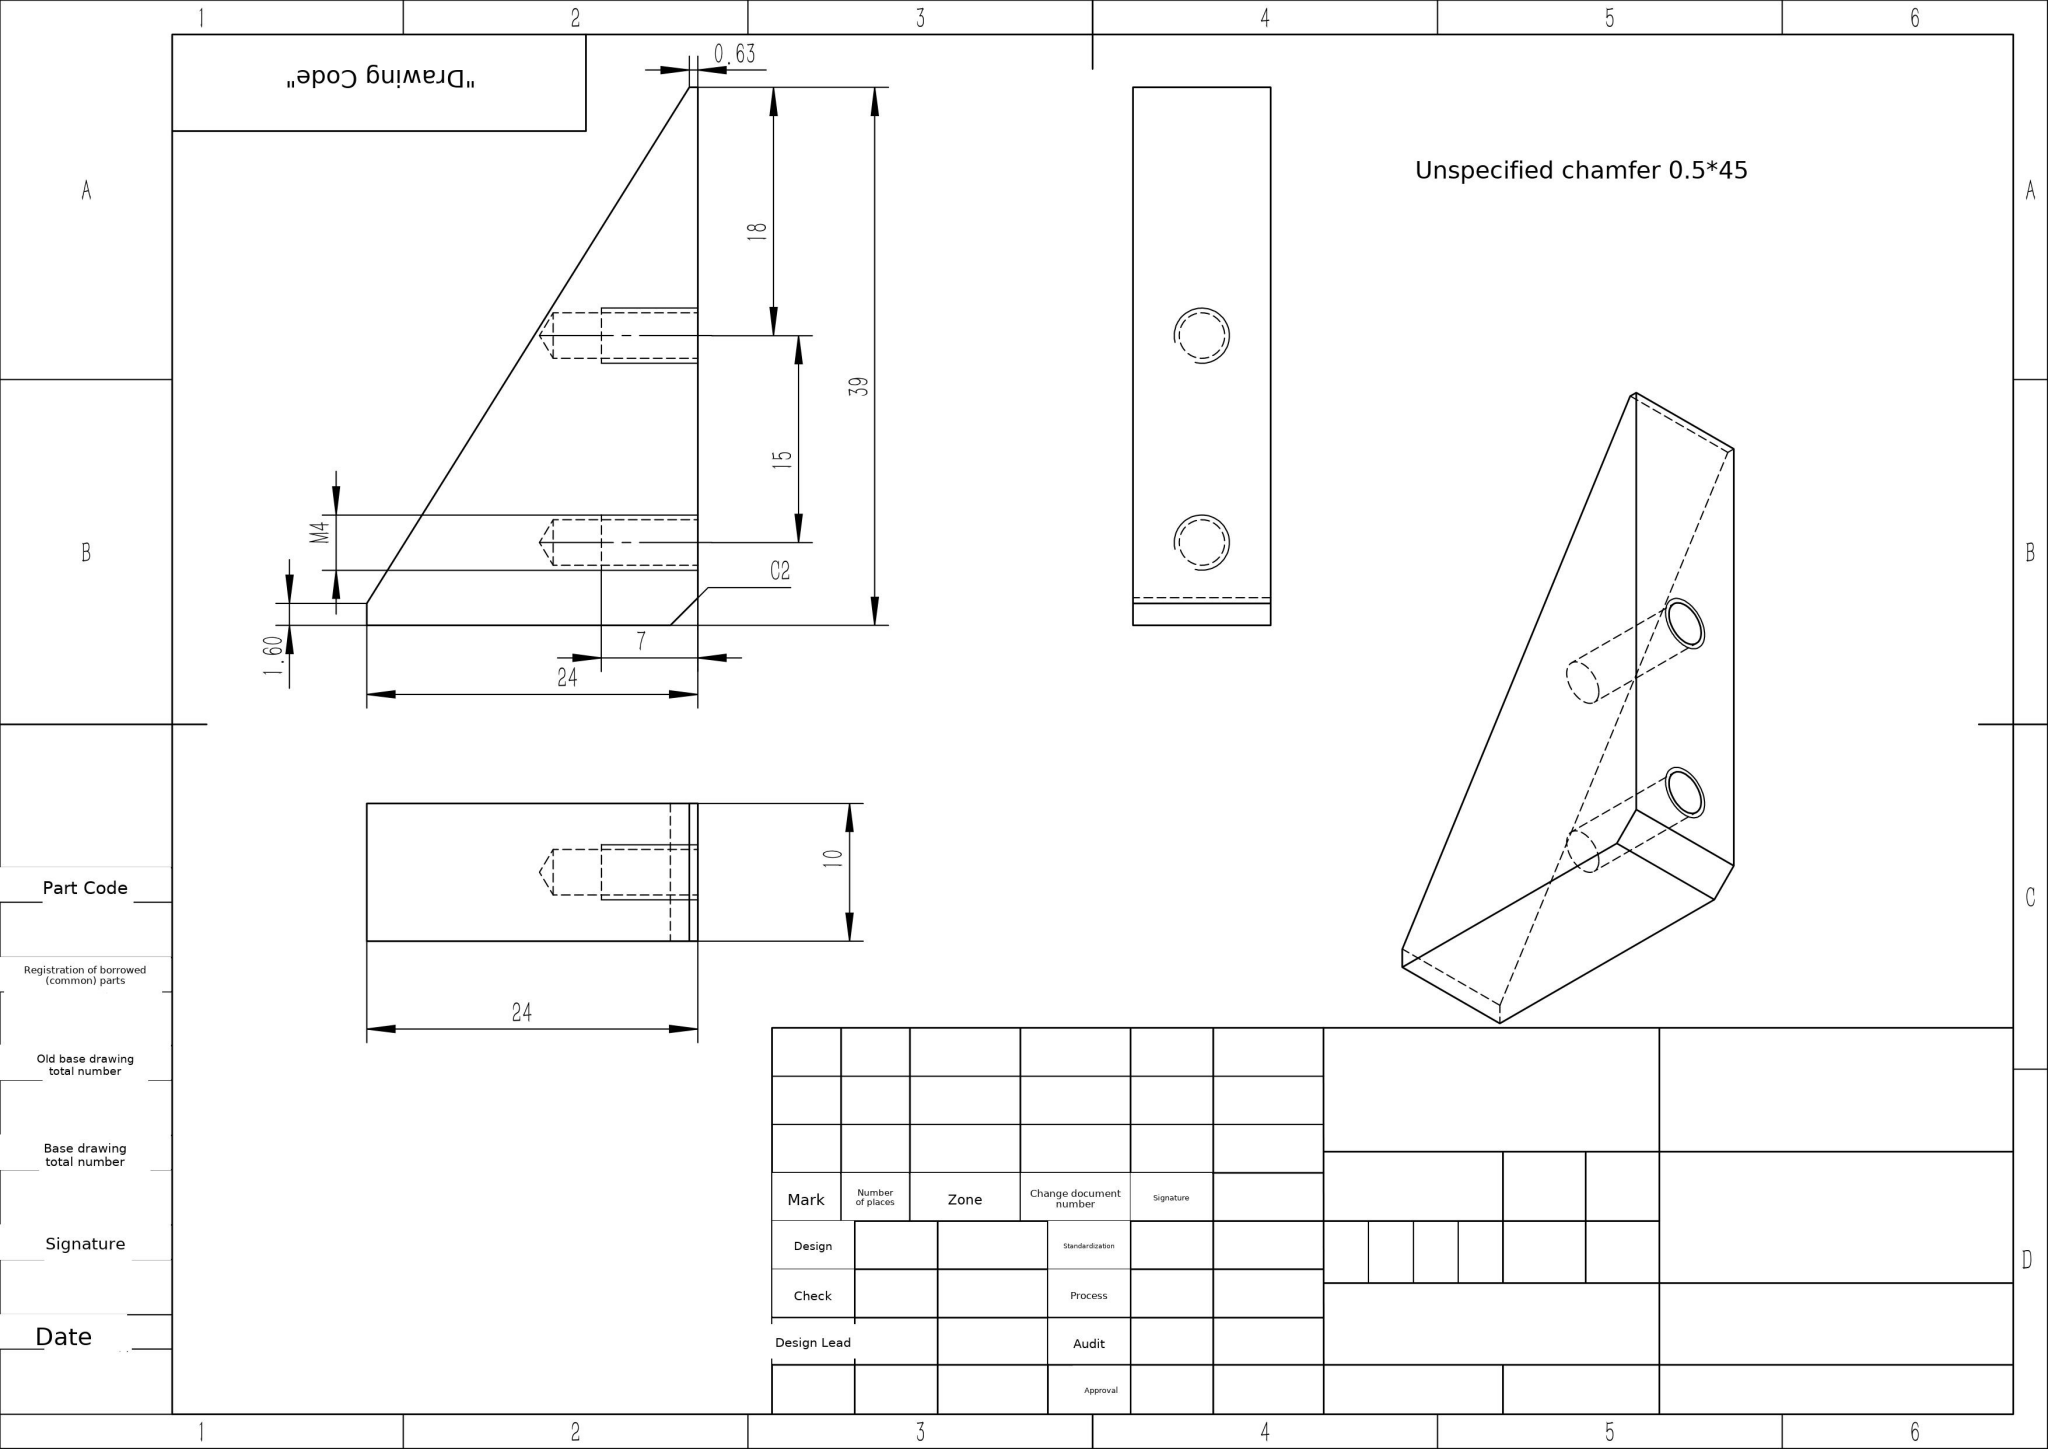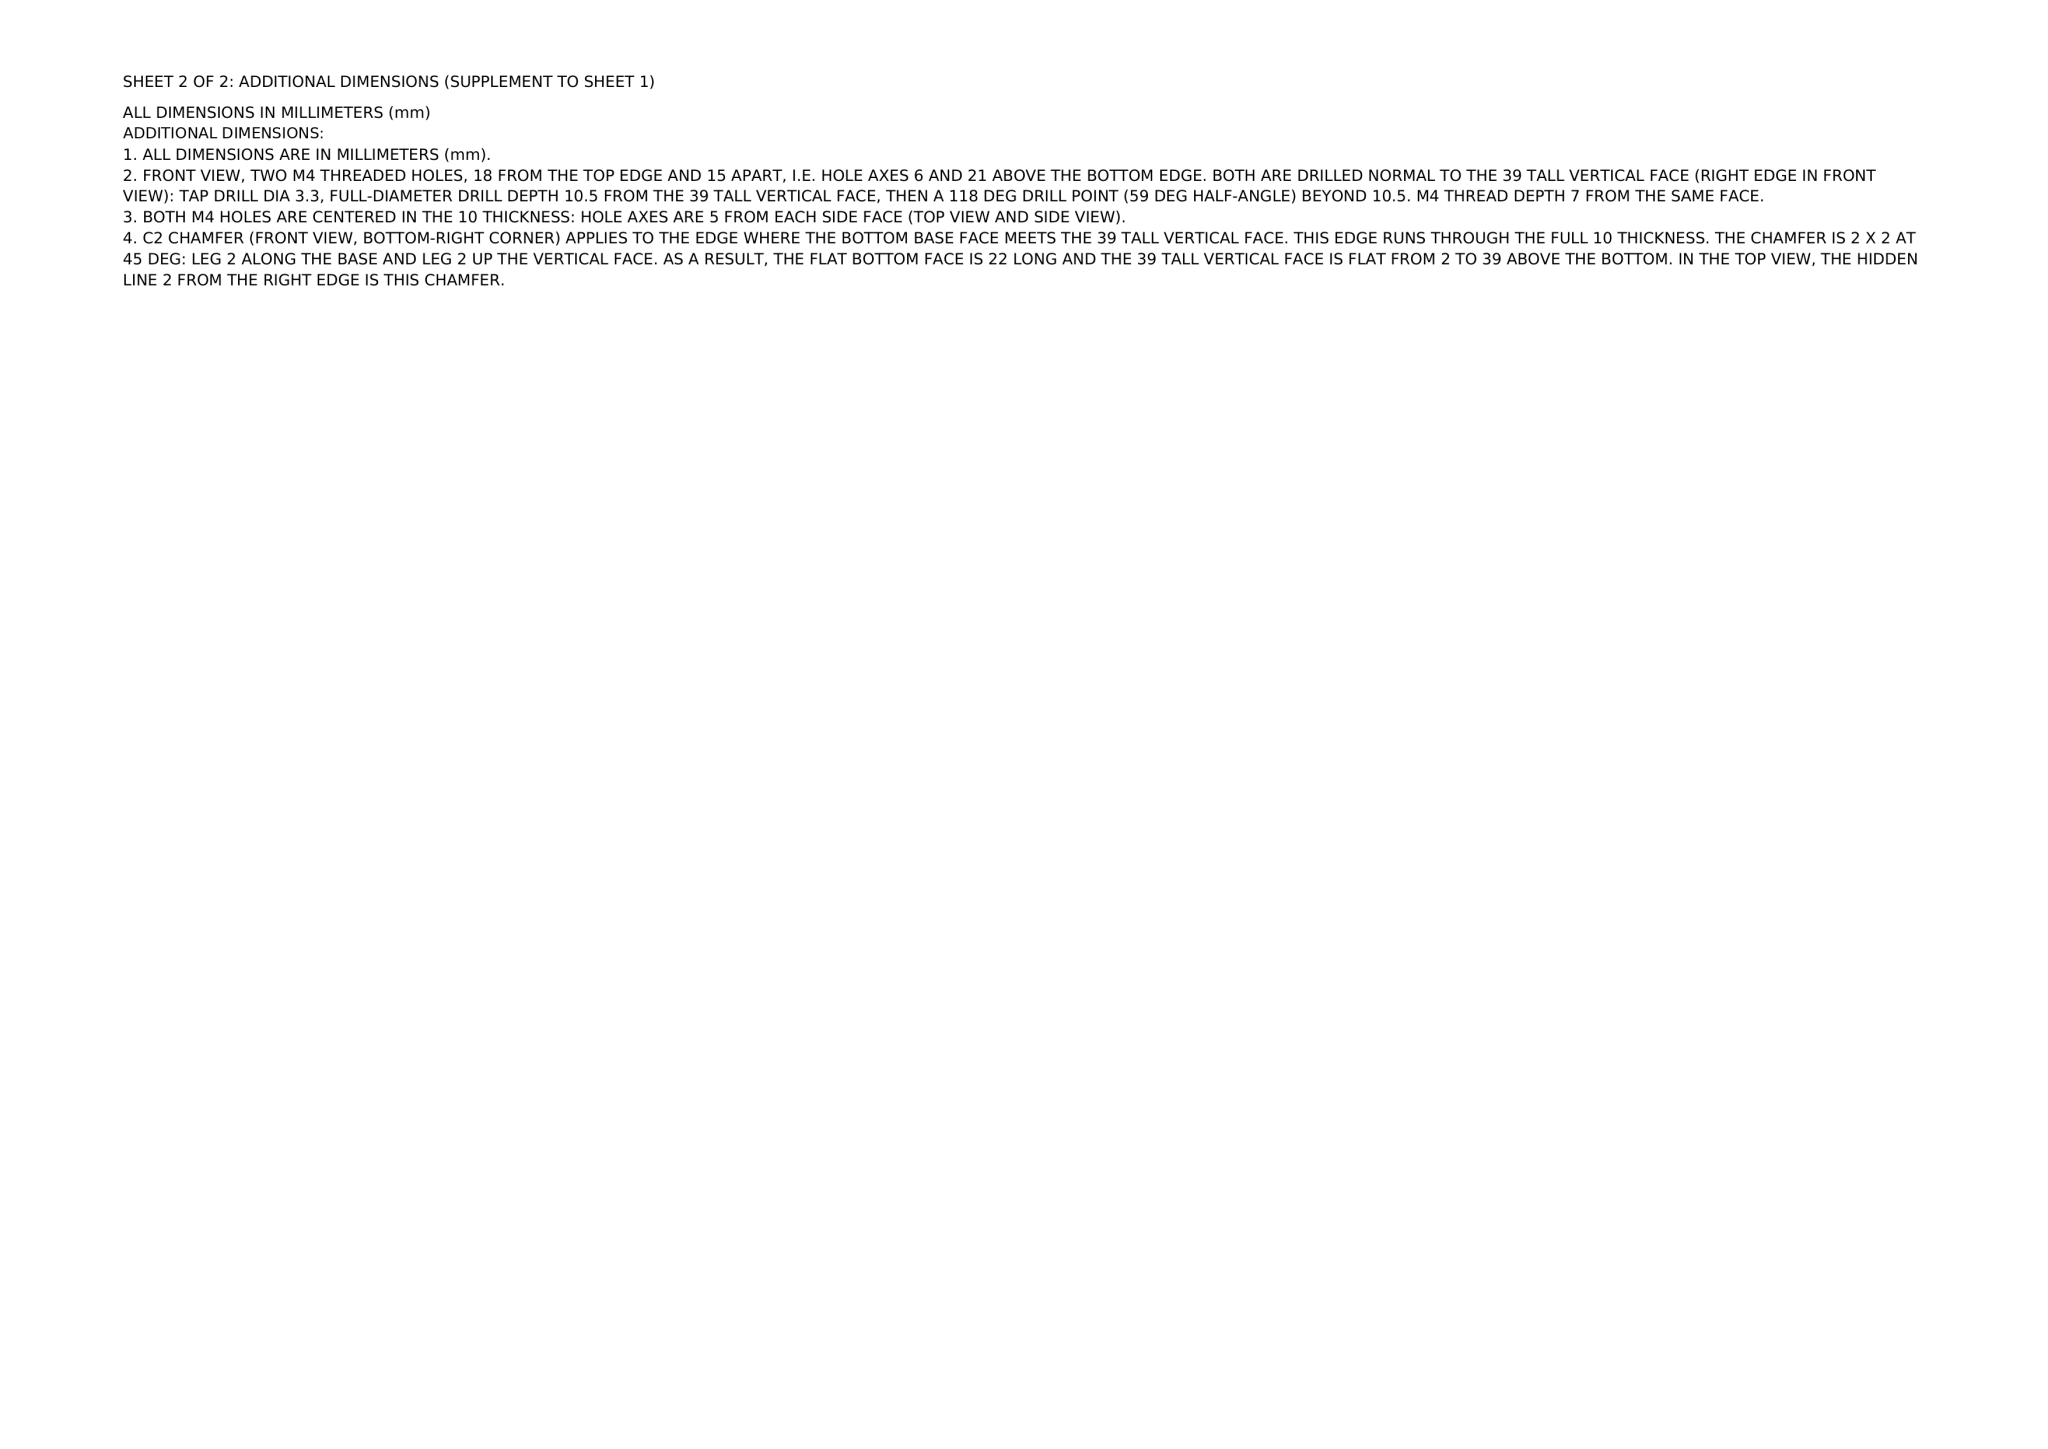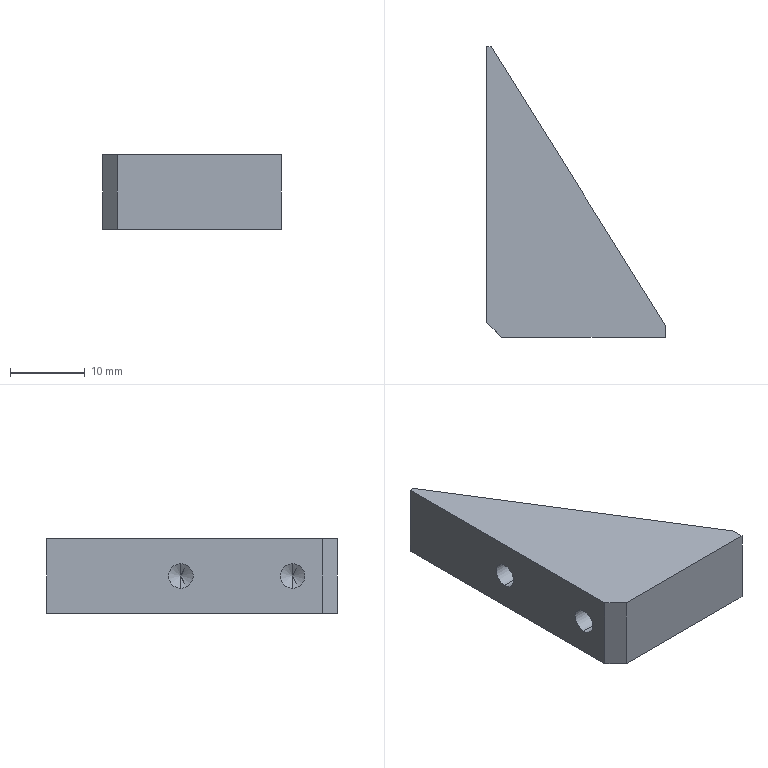Part | NX | mm | Tapered Right-Angle Dual-Bore Bracket | 1 solid | 16 faces | box 24 x 39 x 10 mm | volume 4784 mm3 | plane 8 | cylinder 4 | cone 4 | commonest cylinder face diameters 3.3 x4
STEP:
#1=COLOUR_RGB('',1.,1.,1.);
#2=FILL_AREA_STYLE_COLOUR('',#1);
#3=FILL_AREA_STYLE('',(#2));
#4=SURFACE_STYLE_FILL_AREA(#3);
#5=SURFACE_SIDE_STYLE('',(#4));
#6=SURFACE_STYLE_USAGE(.BOTH.,#5);
#7=PRESENTATION_STYLE_ASSIGNMENT((#6));
#8=CARTESIAN_POINT('',(10.5,6.,3.35));
#9=VERTEX_POINT('',#8);
#10=CARTESIAN_POINT('',(10.5,6.,6.65));
#11=VERTEX_POINT('',#10);
#12=CARTESIAN_POINT('',(10.5,6.,5.));
#13=DIRECTION('',(-1.,0.,0.));
#14=DIRECTION('',(0.,0.,1.));
#15=AXIS2_PLACEMENT_3D('',#12,#13,#14);
#16=CIRCLE('',#15,1.65);
#17=EDGE_CURVE('',#9,#11,#16,.T.);
#18=ORIENTED_EDGE('',*,*,#17,.F.);
#19=CARTESIAN_POINT('',(-0.,6.,3.35));
#20=VERTEX_POINT('',#19);
#21=CARTESIAN_POINT('',(0.,6.,3.35));
#22=DIRECTION('',(-1.,0.,0.));
#23=VECTOR('',#22,1000.);
#24=LINE('',#21,#23);
#25=EDGE_CURVE('',#9,#20,#24,.T.);
#26=ORIENTED_EDGE('',*,*,#25,.T.);
#27=CARTESIAN_POINT('',(-0.,6.,6.65));
#28=VERTEX_POINT('',#27);
#29=CARTESIAN_POINT('',(-0.,6.,5.));
#30=DIRECTION('',(-1.,0.,0.));
#31=DIRECTION('',(0.,0.,1.));
#32=AXIS2_PLACEMENT_3D('',#29,#30,#31);
#33=CIRCLE('',#32,1.65);
#34=EDGE_CURVE('',#20,#28,#33,.T.);
#35=ORIENTED_EDGE('',*,*,#34,.T.);
#36=CARTESIAN_POINT('',(0.,6.,6.65));
#37=DIRECTION('',(-1.,0.,0.));
#38=VECTOR('',#37,1000.);
#39=LINE('',#36,#38);
#40=EDGE_CURVE('',#11,#28,#39,.T.);
#41=ORIENTED_EDGE('',*,*,#40,.F.);
#42=EDGE_LOOP('',(#18,#26,#35,#41));
#43=FACE_OUTER_BOUND('',#42,.T.);
#44=CARTESIAN_POINT('',(0.,6.,5.));
#45=DIRECTION('',(-1.,0.,0.));
#46=DIRECTION('',(0.,0.,1.));
#47=AXIS2_PLACEMENT_3D('',#44,#45,#46);
#48=CYLINDRICAL_SURFACE('',#47,1.65);
#49=ADVANCED_FACE('',(#43),#48,.F.);
#50=STYLED_ITEM('',(#7),#49);
#51=PRESENTATION_LAYER_ASSIGNMENT('','',(#50));
#52=COLOUR_RGB('',1.,1.,1.);
#53=FILL_AREA_STYLE_COLOUR('',#52);
#54=FILL_AREA_STYLE('',(#53));
#55=SURFACE_STYLE_FILL_AREA(#54);
#56=SURFACE_SIDE_STYLE('',(#55));
#57=SURFACE_STYLE_USAGE(.BOTH.,#56);
#58=PRESENTATION_STYLE_ASSIGNMENT((#57));
#59=CARTESIAN_POINT('',(11.491,6.,5.));
#60=VERTEX_POINT('',#59);
#61=CARTESIAN_POINT('',(10.5,6.,6.65));
#62=DIRECTION('',(-0.515,0.,0.8572));
#63=VECTOR('',#62,1000.);
#64=LINE('',#61,#63);
#65=EDGE_CURVE('',#60,#11,#64,.T.);
#66=ORIENTED_EDGE('',*,*,#65,.F.);
#67=CARTESIAN_POINT('',(10.5,6.,3.35));
#68=DIRECTION('',(-0.515,0.,-0.8572));
#69=VECTOR('',#68,1000.);
#70=LINE('',#67,#69);
#71=EDGE_CURVE('',#60,#9,#70,.T.);
#72=ORIENTED_EDGE('',*,*,#71,.T.);
#73=ORIENTED_EDGE('',*,*,#17,.T.);
#74=EDGE_LOOP('',(#66,#72,#73));
#75=FACE_OUTER_BOUND('',#74,.T.);
#76=CARTESIAN_POINT('',(10.5,6.,5.));
#77=DIRECTION('',(-1.,0.,0.));
#78=DIRECTION('',(0.,0.,1.));
#79=AXIS2_PLACEMENT_3D('',#76,#77,#78);
#80=CONICAL_SURFACE('',#79,1.65,1.03);
#81=ADVANCED_FACE('',(#75),#80,.F.);
#82=CARTESIAN_POINT('',(10.5,21.,3.35));
#83=VERTEX_POINT('',#82);
#84=CARTESIAN_POINT('',(10.5,21.,6.65));
#85=VERTEX_POINT('',#84);
#86=CARTESIAN_POINT('',(10.5,21.,5.));
#87=DIRECTION('',(-1.,0.,0.));
#88=DIRECTION('',(0.,0.,1.));
#89=AXIS2_PLACEMENT_3D('',#86,#87,#88);
#90=CIRCLE('',#89,1.65);
#91=EDGE_CURVE('',#83,#85,#90,.T.);
#92=ORIENTED_EDGE('',*,*,#91,.F.);
#93=CARTESIAN_POINT('',(-0.,21.,3.35));
#94=VERTEX_POINT('',#93);
#95=CARTESIAN_POINT('',(0.,21.,3.35));
#96=DIRECTION('',(-1.,0.,0.));
#97=VECTOR('',#96,1000.);
#98=LINE('',#95,#97);
#99=EDGE_CURVE('',#83,#94,#98,.T.);
#100=ORIENTED_EDGE('',*,*,#99,.T.);
#101=CARTESIAN_POINT('',(-0.,21.,6.65));
#102=VERTEX_POINT('',#101);
#103=CARTESIAN_POINT('',(-0.,21.,5.));
#104=DIRECTION('',(-1.,0.,0.));
#105=DIRECTION('',(0.,0.,1.));
#106=AXIS2_PLACEMENT_3D('',#103,#104,#105);
#107=CIRCLE('',#106,1.65);
#108=EDGE_CURVE('',#94,#102,#107,.T.);
#109=ORIENTED_EDGE('',*,*,#108,.T.);
#110=CARTESIAN_POINT('',(0.,21.,6.65));
#111=DIRECTION('',(-1.,0.,0.));
#112=VECTOR('',#111,1000.);
#113=LINE('',#110,#112);
#114=EDGE_CURVE('',#85,#102,#113,.T.);
#115=ORIENTED_EDGE('',*,*,#114,.F.);
#116=EDGE_LOOP('',(#92,#100,#109,#115));
#117=FACE_OUTER_BOUND('',#116,.T.);
#118=CARTESIAN_POINT('',(0.,21.,5.));
#119=DIRECTION('',(-1.,0.,0.));
#120=DIRECTION('',(0.,0.,1.));
#121=AXIS2_PLACEMENT_3D('',#118,#119,#120);
#122=CYLINDRICAL_SURFACE('',#121,1.65);
#123=ADVANCED_FACE('',(#117),#122,.F.);
#124=CARTESIAN_POINT('',(11.491,21.,5.));
#125=VERTEX_POINT('',#124);
#126=CARTESIAN_POINT('',(10.5,21.,6.65));
#127=DIRECTION('',(-0.515,0.,0.8572));
#128=VECTOR('',#127,1000.);
#129=LINE('',#126,#128);
#130=EDGE_CURVE('',#125,#85,#129,.T.);
#131=ORIENTED_EDGE('',*,*,#130,.F.);
#132=CARTESIAN_POINT('',(10.5,21.,3.35));
#133=DIRECTION('',(-0.515,0.,-0.8572));
#134=VECTOR('',#133,1000.);
#135=LINE('',#132,#134);
#136=EDGE_CURVE('',#125,#83,#135,.T.);
#137=ORIENTED_EDGE('',*,*,#136,.T.);
#138=ORIENTED_EDGE('',*,*,#91,.T.);
#139=EDGE_LOOP('',(#131,#137,#138));
#140=FACE_OUTER_BOUND('',#139,.T.);
#141=CARTESIAN_POINT('',(10.5,21.,5.));
#142=DIRECTION('',(-1.,0.,0.));
#143=DIRECTION('',(0.,0.,1.));
#144=AXIS2_PLACEMENT_3D('',#141,#142,#143);
#145=CONICAL_SURFACE('',#144,1.65,1.03);
#146=ADVANCED_FACE('',(#140),#145,.F.);
#147=CARTESIAN_POINT('',(2.,0.,10.));
#148=VERTEX_POINT('',#147);
#149=CARTESIAN_POINT('',(24.,0.,10.));
#150=VERTEX_POINT('',#149);
#151=CARTESIAN_POINT('',(0.,0.,10.));
#152=DIRECTION('',(1.,0.,0.));
#153=VECTOR('',#152,1000.);
#154=LINE('',#151,#153);
#155=EDGE_CURVE('',#148,#150,#154,.T.);
#156=ORIENTED_EDGE('',*,*,#155,.F.);
#157=CARTESIAN_POINT('',(2.,0.,0.));
#158=VERTEX_POINT('',#157);
#159=CARTESIAN_POINT('',(2.,0.,10.));
#160=DIRECTION('',(0.,0.,-1.));
#161=VECTOR('',#160,1000.);
#162=LINE('',#159,#161);
#163=EDGE_CURVE('',#148,#158,#162,.T.);
#164=ORIENTED_EDGE('',*,*,#163,.T.);
#165=CARTESIAN_POINT('',(24.,0.,0.));
#166=VERTEX_POINT('',#165);
#167=CARTESIAN_POINT('',(0.,0.,0.));
#168=DIRECTION('',(1.,0.,0.));
#169=VECTOR('',#168,1000.);
#170=LINE('',#167,#169);
#171=EDGE_CURVE('',#158,#166,#170,.T.);
#172=ORIENTED_EDGE('',*,*,#171,.T.);
#173=CARTESIAN_POINT('',(24.,0.,10.));
#174=DIRECTION('',(0.,0.,-1.));
#175=VECTOR('',#174,1000.);
#176=LINE('',#173,#175);
#177=EDGE_CURVE('',#150,#166,#176,.T.);
#178=ORIENTED_EDGE('',*,*,#177,.F.);
#179=EDGE_LOOP('',(#156,#164,#172,#178));
#180=FACE_OUTER_BOUND('',#179,.T.);
#181=CARTESIAN_POINT('',(0.,0.,10.));
#182=DIRECTION('',(0.,1.,0.));
#183=DIRECTION('',(0.,0.,1.));
#184=AXIS2_PLACEMENT_3D('',#181,#182,#183);
#185=PLANE('',#184);
#186=ADVANCED_FACE('',(#180),#185,.F.);
#187=CARTESIAN_POINT('',(24.,1.6,10.));
#188=VERTEX_POINT('',#187);
#189=CARTESIAN_POINT('',(0.625,39.,10.));
#190=VERTEX_POINT('',#189);
#191=CARTESIAN_POINT('',(0.,40.,10.));
#192=DIRECTION('',(-0.53,0.848,0.));
#193=VECTOR('',#192,1000.);
#194=LINE('',#191,#193);
#195=EDGE_CURVE('',#188,#190,#194,.T.);
#196=ORIENTED_EDGE('',*,*,#195,.F.);
#197=CARTESIAN_POINT('',(24.,1.6,0.));
#198=VERTEX_POINT('',#197);
#199=CARTESIAN_POINT('',(24.,1.6,10.));
#200=DIRECTION('',(0.,0.,-1.));
#201=VECTOR('',#200,1000.);
#202=LINE('',#199,#201);
#203=EDGE_CURVE('',#188,#198,#202,.T.);
#204=ORIENTED_EDGE('',*,*,#203,.T.);
#205=CARTESIAN_POINT('',(0.625,39.,0.));
#206=VERTEX_POINT('',#205);
#207=CARTESIAN_POINT('',(0.,40.,0.));
#208=DIRECTION('',(-0.53,0.848,0.));
#209=VECTOR('',#208,1000.);
#210=LINE('',#207,#209);
#211=EDGE_CURVE('',#198,#206,#210,.T.);
#212=ORIENTED_EDGE('',*,*,#211,.T.);
#213=CARTESIAN_POINT('',(0.625,39.,10.));
#214=DIRECTION('',(0.,0.,1.));
#215=VECTOR('',#214,1000.);
#216=LINE('',#213,#215);
#217=EDGE_CURVE('',#206,#190,#216,.T.);
#218=ORIENTED_EDGE('',*,*,#217,.T.);
#219=EDGE_LOOP('',(#196,#204,#212,#218));
#220=FACE_OUTER_BOUND('',#219,.T.);
#221=CARTESIAN_POINT('',(0.,40.,10.));
#222=DIRECTION('',(-0.848,-0.53,0.));
#223=DIRECTION('',(0.53,-0.848,0.));
#224=AXIS2_PLACEMENT_3D('',#221,#222,#223);
#225=PLANE('',#224);
#226=ADVANCED_FACE('',(#220),#225,.F.);
#227=CARTESIAN_POINT('',(-0.,6.,5.));
#228=DIRECTION('',(-1.,0.,0.));
#229=DIRECTION('',(0.,0.,1.));
#230=AXIS2_PLACEMENT_3D('',#227,#228,#229);
#231=CIRCLE('',#230,1.65);
#232=EDGE_CURVE('',#28,#20,#231,.T.);
#233=ORIENTED_EDGE('',*,*,#232,.F.);
#234=ORIENTED_EDGE('',*,*,#34,.F.);
#235=EDGE_LOOP('',(#233,#234));
#236=FACE_BOUND('',#235,.T.);
#237=CARTESIAN_POINT('',(-0.,21.,5.));
#238=DIRECTION('',(-1.,0.,0.));
#239=DIRECTION('',(0.,0.,1.));
#240=AXIS2_PLACEMENT_3D('',#237,#238,#239);
#241=CIRCLE('',#240,1.65);
#242=EDGE_CURVE('',#102,#94,#241,.T.);
#243=ORIENTED_EDGE('',*,*,#242,.F.);
#244=ORIENTED_EDGE('',*,*,#108,.F.);
#245=EDGE_LOOP('',(#243,#244));
#246=FACE_BOUND('',#245,.T.);
#247=CARTESIAN_POINT('',(-0.,39.,0.));
#248=VERTEX_POINT('',#247);
#249=CARTESIAN_POINT('',(0.,2.,0.));
#250=VERTEX_POINT('',#249);
#251=CARTESIAN_POINT('',(0.,0.,0.));
#252=DIRECTION('',(0.,-1.,0.));
#253=VECTOR('',#252,1000.);
#254=LINE('',#251,#253);
#255=EDGE_CURVE('',#248,#250,#254,.T.);
#256=ORIENTED_EDGE('',*,*,#255,.T.);
#257=CARTESIAN_POINT('',(0.,2.,10.));
#258=VERTEX_POINT('',#257);
#259=CARTESIAN_POINT('',(0.,2.,10.));
#260=DIRECTION('',(0.,0.,1.));
#261=VECTOR('',#260,1000.);
#262=LINE('',#259,#261);
#263=EDGE_CURVE('',#250,#258,#262,.T.);
#264=ORIENTED_EDGE('',*,*,#263,.T.);
#265=CARTESIAN_POINT('',(-0.,39.,10.));
#266=VERTEX_POINT('',#265);
#267=CARTESIAN_POINT('',(0.,0.,10.));
#268=DIRECTION('',(0.,-1.,0.));
#269=VECTOR('',#268,1000.);
#270=LINE('',#267,#269);
#271=EDGE_CURVE('',#266,#258,#270,.T.);
#272=ORIENTED_EDGE('',*,*,#271,.F.);
#273=CARTESIAN_POINT('',(-0.,39.,10.));
#274=DIRECTION('',(0.,0.,-1.));
#275=VECTOR('',#274,1000.);
#276=LINE('',#273,#275);
#277=EDGE_CURVE('',#266,#248,#276,.T.);
#278=ORIENTED_EDGE('',*,*,#277,.T.);
#279=EDGE_LOOP('',(#256,#264,#272,#278));
#280=FACE_OUTER_BOUND('',#279,.T.);
#281=CARTESIAN_POINT('',(0.,0.,10.));
#282=DIRECTION('',(1.,0.,0.));
#283=DIRECTION('',(0.,0.,-1.));
#284=AXIS2_PLACEMENT_3D('',#281,#282,#283);
#285=PLANE('',#284);
#286=ADVANCED_FACE('',(#236,#246,#280),#285,.F.);
#287=ORIENTED_EDGE('',*,*,#271,.T.);
#288=CARTESIAN_POINT('',(1.,1.,10.));
#289=DIRECTION('',(0.7071,-0.7071,0.));
#290=VECTOR('',#289,1000.);
#291=LINE('',#288,#290);
#292=EDGE_CURVE('',#258,#148,#291,.T.);
#293=ORIENTED_EDGE('',*,*,#292,.T.);
#294=ORIENTED_EDGE('',*,*,#155,.T.);
#295=CARTESIAN_POINT('',(24.,0.,10.));
#296=DIRECTION('',(0.,1.,0.));
#297=VECTOR('',#296,1000.);
#298=LINE('',#295,#297);
#299=EDGE_CURVE('',#150,#188,#298,.T.);
#300=ORIENTED_EDGE('',*,*,#299,.T.);
#301=ORIENTED_EDGE('',*,*,#195,.T.);
#302=CARTESIAN_POINT('',(-0.,39.,10.));
#303=DIRECTION('',(-1.,0.,0.));
#304=VECTOR('',#303,1000.);
#305=LINE('',#302,#304);
#306=EDGE_CURVE('',#190,#266,#305,.T.);
#307=ORIENTED_EDGE('',*,*,#306,.T.);
#308=EDGE_LOOP('',(#287,#293,#294,#300,#301,#307));
#309=FACE_OUTER_BOUND('',#308,.T.);
#310=CARTESIAN_POINT('',(0.,0.,10.));
#311=DIRECTION('',(0.,0.,1.));
#312=DIRECTION('',(1.,0.,0.));
#313=AXIS2_PLACEMENT_3D('',#310,#311,#312);
#314=PLANE('',#313);
#315=ADVANCED_FACE('',(#309),#314,.T.);
#316=ORIENTED_EDGE('',*,*,#171,.F.);
#317=CARTESIAN_POINT('',(2.,0.,0.));
#318=DIRECTION('',(-0.7071,0.7071,0.));
#319=VECTOR('',#318,1000.);
#320=LINE('',#317,#319);
#321=EDGE_CURVE('',#158,#250,#320,.T.);
#322=ORIENTED_EDGE('',*,*,#321,.T.);
#323=ORIENTED_EDGE('',*,*,#255,.F.);
#324=CARTESIAN_POINT('',(0.,39.,0.));
#325=DIRECTION('',(1.,0.,0.));
#326=VECTOR('',#325,1000.);
#327=LINE('',#324,#326);
#328=EDGE_CURVE('',#248,#206,#327,.T.);
#329=ORIENTED_EDGE('',*,*,#328,.T.);
#330=ORIENTED_EDGE('',*,*,#211,.F.);
#331=CARTESIAN_POINT('',(24.,0.,0.));
#332=DIRECTION('',(0.,1.,0.));
#333=VECTOR('',#332,1000.);
#334=LINE('',#331,#333);
#335=EDGE_CURVE('',#166,#198,#334,.T.);
#336=ORIENTED_EDGE('',*,*,#335,.F.);
#337=EDGE_LOOP('',(#316,#322,#323,#329,#330,#336));
#338=FACE_OUTER_BOUND('',#337,.T.);
#339=CARTESIAN_POINT('',(0.,0.,0.));
#340=DIRECTION('',(0.,0.,1.));
#341=DIRECTION('',(1.,0.,0.));
#342=AXIS2_PLACEMENT_3D('',#339,#340,#341);
#343=PLANE('',#342);
#344=ADVANCED_FACE('',(#338),#343,.F.);
#345=ORIENTED_EDGE('',*,*,#328,.F.);
#346=ORIENTED_EDGE('',*,*,#277,.F.);
#347=ORIENTED_EDGE('',*,*,#306,.F.);
#348=ORIENTED_EDGE('',*,*,#217,.F.);
#349=EDGE_LOOP('',(#345,#346,#347,#348));
#350=FACE_OUTER_BOUND('',#349,.T.);
#351=CARTESIAN_POINT('',(-0.,39.,10.));
#352=DIRECTION('',(0.,-1.,0.));
#353=DIRECTION('',(0.,0.,-1.));
#354=AXIS2_PLACEMENT_3D('',#351,#352,#353);
#355=PLANE('',#354);
#356=ADVANCED_FACE('',(#350),#355,.F.);
#357=ORIENTED_EDGE('',*,*,#299,.F.);
#358=ORIENTED_EDGE('',*,*,#177,.T.);
#359=ORIENTED_EDGE('',*,*,#335,.T.);
#360=ORIENTED_EDGE('',*,*,#203,.F.);
#361=EDGE_LOOP('',(#357,#358,#359,#360));
#362=FACE_OUTER_BOUND('',#361,.T.);
#363=CARTESIAN_POINT('',(24.,0.,10.));
#364=DIRECTION('',(-1.,0.,0.));
#365=DIRECTION('',(0.,0.,1.));
#366=AXIS2_PLACEMENT_3D('',#363,#364,#365);
#367=PLANE('',#366);
#368=ADVANCED_FACE('',(#362),#367,.F.);
#369=ORIENTED_EDGE('',*,*,#292,.F.);
#370=ORIENTED_EDGE('',*,*,#263,.F.);
#371=ORIENTED_EDGE('',*,*,#321,.F.);
#372=ORIENTED_EDGE('',*,*,#163,.F.);
#373=EDGE_LOOP('',(#369,#370,#371,#372));
#374=FACE_OUTER_BOUND('',#373,.T.);
#375=CARTESIAN_POINT('',(2.,0.,10.));
#376=DIRECTION('',(0.7071,0.7071,0.));
#377=DIRECTION('',(0.,0.,-1.));
#378=AXIS2_PLACEMENT_3D('',#375,#376,#377);
#379=PLANE('',#378);
#380=ADVANCED_FACE('',(#374),#379,.F.);
#381=ORIENTED_EDGE('',*,*,#136,.F.);
#382=ORIENTED_EDGE('',*,*,#130,.T.);
#383=CARTESIAN_POINT('',(10.5,21.,5.));
#384=DIRECTION('',(-1.,0.,0.));
#385=DIRECTION('',(0.,0.,1.));
#386=AXIS2_PLACEMENT_3D('',#383,#384,#385);
#387=CIRCLE('',#386,1.65);
#388=EDGE_CURVE('',#85,#83,#387,.T.);
#389=ORIENTED_EDGE('',*,*,#388,.T.);
#390=EDGE_LOOP('',(#381,#382,#389));
#391=FACE_OUTER_BOUND('',#390,.T.);
#392=CARTESIAN_POINT('',(10.5,21.,5.));
#393=DIRECTION('',(-1.,0.,0.));
#394=DIRECTION('',(0.,0.,1.));
#395=AXIS2_PLACEMENT_3D('',#392,#393,#394);
#396=CONICAL_SURFACE('',#395,1.65,1.03);
#397=ADVANCED_FACE('',(#391),#396,.F.);
#398=ORIENTED_EDGE('',*,*,#99,.F.);
#399=ORIENTED_EDGE('',*,*,#388,.F.);
#400=ORIENTED_EDGE('',*,*,#114,.T.);
#401=ORIENTED_EDGE('',*,*,#242,.T.);
#402=EDGE_LOOP('',(#398,#399,#400,#401));
#403=FACE_OUTER_BOUND('',#402,.T.);
#404=CARTESIAN_POINT('',(0.,21.,5.));
#405=DIRECTION('',(-1.,0.,0.));
#406=DIRECTION('',(0.,0.,1.));
#407=AXIS2_PLACEMENT_3D('',#404,#405,#406);
#408=CYLINDRICAL_SURFACE('',#407,1.65);
#409=ADVANCED_FACE('',(#403),#408,.F.);
#410=ORIENTED_EDGE('',*,*,#71,.F.);
#411=ORIENTED_EDGE('',*,*,#65,.T.);
#412=CARTESIAN_POINT('',(10.5,6.,5.));
#413=DIRECTION('',(-1.,0.,0.));
#414=DIRECTION('',(0.,0.,1.));
#415=AXIS2_PLACEMENT_3D('',#412,#413,#414);
#416=CIRCLE('',#415,1.65);
#417=EDGE_CURVE('',#11,#9,#416,.T.);
#418=ORIENTED_EDGE('',*,*,#417,.T.);
#419=EDGE_LOOP('',(#410,#411,#418));
#420=FACE_OUTER_BOUND('',#419,.T.);
#421=CARTESIAN_POINT('',(10.5,6.,5.));
#422=DIRECTION('',(-1.,0.,0.));
#423=DIRECTION('',(0.,0.,1.));
#424=AXIS2_PLACEMENT_3D('',#421,#422,#423);
#425=CONICAL_SURFACE('',#424,1.65,1.03);
#426=ADVANCED_FACE('',(#420),#425,.F.);
#427=ORIENTED_EDGE('',*,*,#25,.F.);
#428=ORIENTED_EDGE('',*,*,#417,.F.);
#429=ORIENTED_EDGE('',*,*,#40,.T.);
#430=ORIENTED_EDGE('',*,*,#232,.T.);
#431=EDGE_LOOP('',(#427,#428,#429,#430));
#432=FACE_OUTER_BOUND('',#431,.T.);
#433=CARTESIAN_POINT('',(0.,6.,5.));
#434=DIRECTION('',(-1.,0.,0.));
#435=DIRECTION('',(0.,0.,1.));
#436=AXIS2_PLACEMENT_3D('',#433,#434,#435);
#437=CYLINDRICAL_SURFACE('',#436,1.65);
#438=ADVANCED_FACE('',(#432),#437,.F.);
#439=CLOSED_SHELL('',(#49,#81,#123,#146,#186,#226,#286,#315,#344,#356,#368,#380,#397,#409,#426,#438));
#440=MANIFOLD_SOLID_BREP('',#439);
#441=STYLED_ITEM('',(#58),#440);
#442=PRESENTATION_LAYER_ASSIGNMENT('','',(#441));
#443=COLOUR_RGB('',1.,1.,1.);
#444=FILL_AREA_STYLE_COLOUR('',#443);
#445=FILL_AREA_STYLE('',(#444));
#446=SURFACE_STYLE_FILL_AREA(#445);
#447=SURFACE_SIDE_STYLE('',(#446));
#448=SURFACE_STYLE_USAGE(.BOTH.,#447);
#449=PRESENTATION_STYLE_ASSIGNMENT((#448));
#450=CARTESIAN_POINT('',(0.,0.,0.));
#451=DIRECTION('',(0.,0.,1.));
#452=DIRECTION('',(1.,0.,0.));
#453=AXIS2_PLACEMENT_3D('',#450,#451,#452);
#454=(LENGTH_UNIT()NAMED_UNIT(*)SI_UNIT(.MILLI.,.METRE.));
#455=UNCERTAINTY_MEASURE_WITH_UNIT(LENGTH_MEASURE(0.00001),#454,'','');
#456=(NAMED_UNIT(*)PLANE_ANGLE_UNIT()SI_UNIT($,.RADIAN.));
#457=(NAMED_UNIT(*)SI_UNIT($,.STERADIAN.)SOLID_ANGLE_UNIT());
#458=(GEOMETRIC_REPRESENTATION_CONTEXT(3)GLOBAL_UNCERTAINTY_ASSIGNED_CONTEXT((#455))GLOBAL_UNIT_ASSIGNED_CONTEXT((#454,#456,#457))REPRESENTATION_CONTEXT('',''));
#459=ADVANCED_BREP_SHAPE_REPRESENTATION('',(#440,#453),#458);
#460=STYLED_ITEM('',(#449),#459);
#461=(LENGTH_UNIT()NAMED_UNIT(*)SI_UNIT(.MILLI.,.METRE.));
#462=UNCERTAINTY_MEASURE_WITH_UNIT(LENGTH_MEASURE(0.00001),#461,'','');
#463=(NAMED_UNIT(*)PLANE_ANGLE_UNIT()SI_UNIT($,.RADIAN.));
#464=(NAMED_UNIT(*)SI_UNIT($,.STERADIAN.)SOLID_ANGLE_UNIT());
#465=(GEOMETRIC_REPRESENTATION_CONTEXT(3)GLOBAL_UNCERTAINTY_ASSIGNED_CONTEXT((#462))GLOBAL_UNIT_ASSIGNED_CONTEXT((#461,#463,#464))REPRESENTATION_CONTEXT('',''));
#466=MECHANICAL_DESIGN_GEOMETRIC_PRESENTATION_REPRESENTATION('',(#460),#465);
#467=COLOUR_RGB('',1.,1.,1.);
#468=FILL_AREA_STYLE_COLOUR('',#467);
#469=FILL_AREA_STYLE('',(#468));
#470=SURFACE_STYLE_FILL_AREA(#469);
#471=SURFACE_SIDE_STYLE('',(#470));
#472=SURFACE_STYLE_USAGE(.BOTH.,#471);
#473=PRESENTATION_STYLE_ASSIGNMENT((#472));
#474=STYLED_ITEM('',(#473),#438);
#475=PRESENTATION_LAYER_ASSIGNMENT('','',(#474));
#476=(LENGTH_UNIT()NAMED_UNIT(*)SI_UNIT(.MILLI.,.METRE.));
#477=UNCERTAINTY_MEASURE_WITH_UNIT(LENGTH_MEASURE(0.00001),#476,'','');
#478=(NAMED_UNIT(*)PLANE_ANGLE_UNIT()SI_UNIT($,.RADIAN.));
#479=(NAMED_UNIT(*)SI_UNIT($,.STERADIAN.)SOLID_ANGLE_UNIT());
#480=(GEOMETRIC_REPRESENTATION_CONTEXT(3)GLOBAL_UNCERTAINTY_ASSIGNED_CONTEXT((#477))GLOBAL_UNIT_ASSIGNED_CONTEXT((#476,#478,#479))REPRESENTATION_CONTEXT('',''));
#481=MECHANICAL_DESIGN_GEOMETRIC_PRESENTATION_REPRESENTATION('',(#50),#480);
#482=COLOUR_RGB('',1.,1.,1.);
#483=FILL_AREA_STYLE_COLOUR('',#482);
#484=FILL_AREA_STYLE('',(#483));
#485=SURFACE_STYLE_FILL_AREA(#484);
#486=SURFACE_SIDE_STYLE('',(#485));
#487=SURFACE_STYLE_USAGE(.BOTH.,#486);
#488=PRESENTATION_STYLE_ASSIGNMENT((#487));
#489=STYLED_ITEM('',(#488),#123);
#490=(LENGTH_UNIT()NAMED_UNIT(*)SI_UNIT(.MILLI.,.METRE.));
#491=UNCERTAINTY_MEASURE_WITH_UNIT(LENGTH_MEASURE(0.00001),#490,'','');
#492=(NAMED_UNIT(*)PLANE_ANGLE_UNIT()SI_UNIT($,.RADIAN.));
#493=(NAMED_UNIT(*)SI_UNIT($,.STERADIAN.)SOLID_ANGLE_UNIT());
#494=(GEOMETRIC_REPRESENTATION_CONTEXT(3)GLOBAL_UNCERTAINTY_ASSIGNED_CONTEXT((#491))GLOBAL_UNIT_ASSIGNED_CONTEXT((#490,#492,#493))REPRESENTATION_CONTEXT('',''));
#495=MECHANICAL_DESIGN_GEOMETRIC_PRESENTATION_REPRESENTATION('',(#489),#494);
#496=COLOUR_RGB('',1.,1.,1.);
#497=FILL_AREA_STYLE_COLOUR('',#496);
#498=FILL_AREA_STYLE('',(#497));
#499=SURFACE_STYLE_FILL_AREA(#498);
#500=SURFACE_SIDE_STYLE('',(#499));
#501=SURFACE_STYLE_USAGE(.BOTH.,#500);
#502=PRESENTATION_STYLE_ASSIGNMENT((#501));
#503=STYLED_ITEM('',(#502),#409);
#504=(LENGTH_UNIT()NAMED_UNIT(*)SI_UNIT(.MILLI.,.METRE.));
#505=UNCERTAINTY_MEASURE_WITH_UNIT(LENGTH_MEASURE(0.00001),#504,'','');
#506=(NAMED_UNIT(*)PLANE_ANGLE_UNIT()SI_UNIT($,.RADIAN.));
#507=(NAMED_UNIT(*)SI_UNIT($,.STERADIAN.)SOLID_ANGLE_UNIT());
#508=(GEOMETRIC_REPRESENTATION_CONTEXT(3)GLOBAL_UNCERTAINTY_ASSIGNED_CONTEXT((#505))GLOBAL_UNIT_ASSIGNED_CONTEXT((#504,#506,#507))REPRESENTATION_CONTEXT('',''));
#509=MECHANICAL_DESIGN_GEOMETRIC_PRESENTATION_REPRESENTATION('',(#503),#508);
#510=PRESENTATION_LAYER_ASSIGNMENT('','',(#503));
#511=(LENGTH_UNIT()NAMED_UNIT(*)SI_UNIT(.MILLI.,.METRE.));
#512=UNCERTAINTY_MEASURE_WITH_UNIT(LENGTH_MEASURE(0.00001),#511,'','');
#513=(NAMED_UNIT(*)PLANE_ANGLE_UNIT()SI_UNIT($,.RADIAN.));
#514=(NAMED_UNIT(*)SI_UNIT($,.STERADIAN.)SOLID_ANGLE_UNIT());
#515=(GEOMETRIC_REPRESENTATION_CONTEXT(3)GLOBAL_UNCERTAINTY_ASSIGNED_CONTEXT((#512))GLOBAL_UNIT_ASSIGNED_CONTEXT((#511,#513,#514))REPRESENTATION_CONTEXT('',''));
#516=MECHANICAL_DESIGN_GEOMETRIC_PRESENTATION_REPRESENTATION('',(#474),#515);
#517=PRESENTATION_LAYER_ASSIGNMENT('','',(#460));
#518=(LENGTH_UNIT()NAMED_UNIT(*)SI_UNIT(.MILLI.,.METRE.));
#519=UNCERTAINTY_MEASURE_WITH_UNIT(LENGTH_MEASURE(0.00001),#518,'','');
#520=(NAMED_UNIT(*)PLANE_ANGLE_UNIT()SI_UNIT($,.RADIAN.));
#521=(NAMED_UNIT(*)SI_UNIT($,.STERADIAN.)SOLID_ANGLE_UNIT());
#522=(GEOMETRIC_REPRESENTATION_CONTEXT(3)GLOBAL_UNCERTAINTY_ASSIGNED_CONTEXT((#519))GLOBAL_UNIT_ASSIGNED_CONTEXT((#518,#520,#521))REPRESENTATION_CONTEXT('',''));
#523=MECHANICAL_DESIGN_GEOMETRIC_PRESENTATION_REPRESENTATION('',(#441),#522);
#524=PRESENTATION_LAYER_ASSIGNMENT('','',(#489));